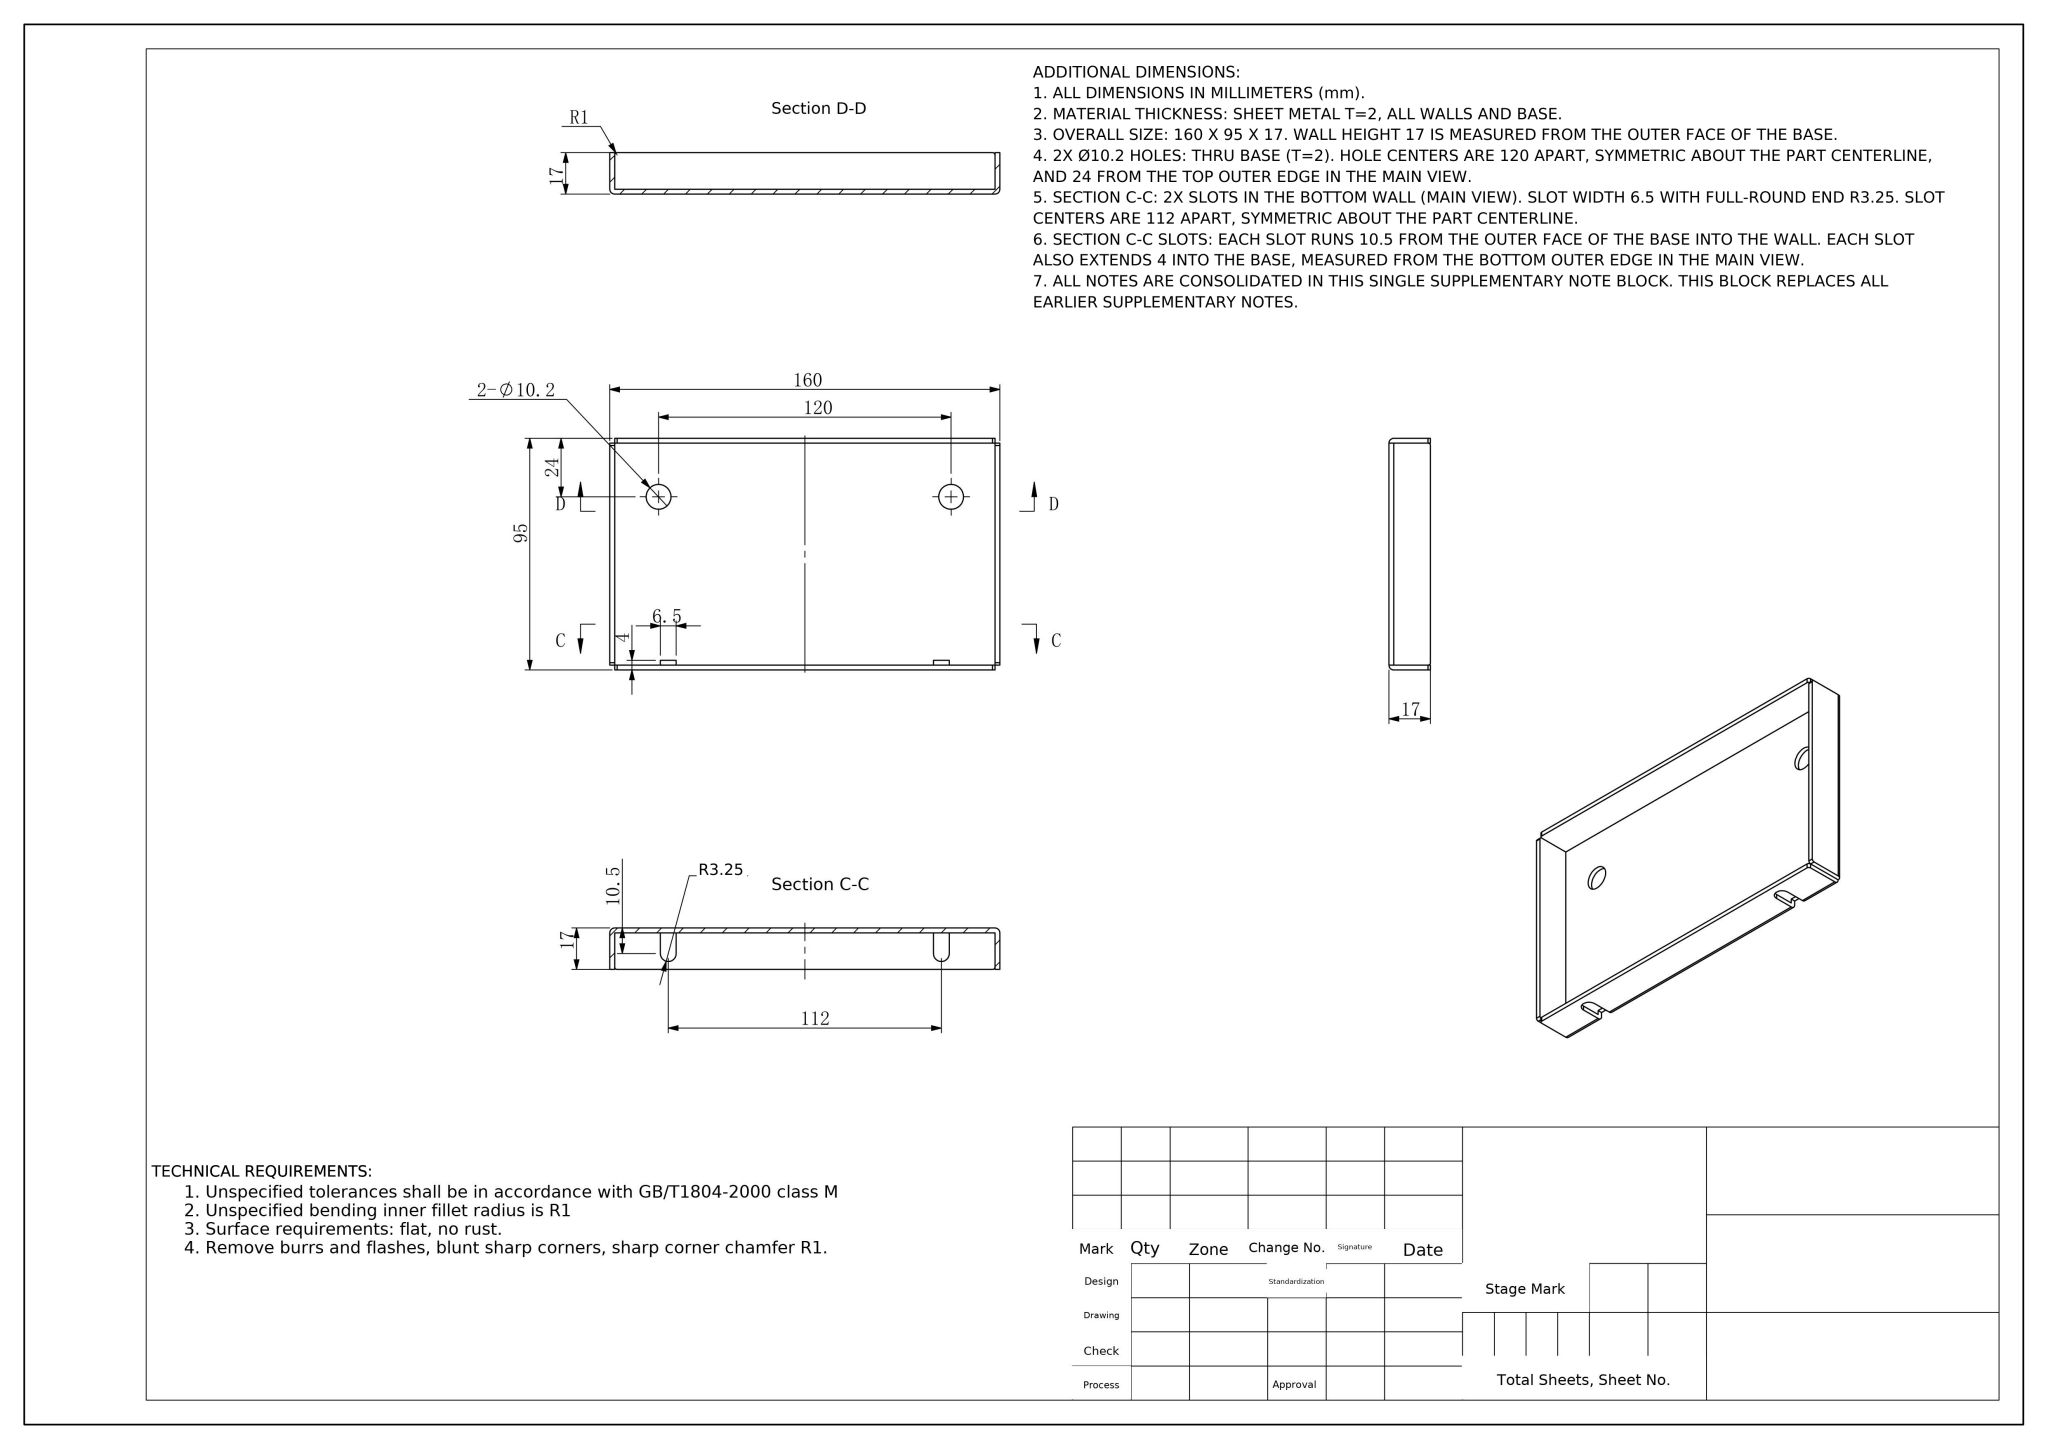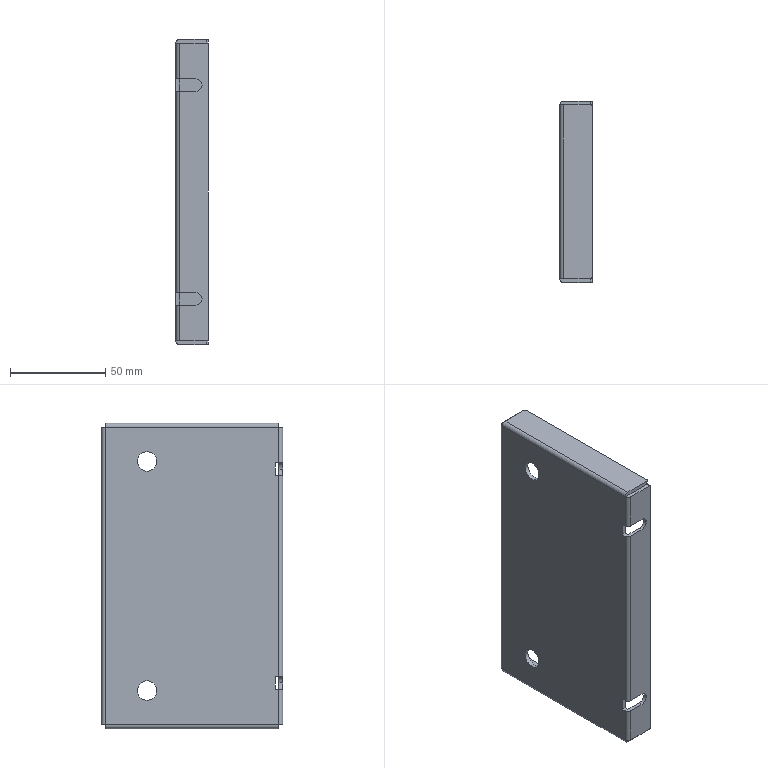Part | NX | mm | 1 solid | 64 faces | box 17 x 95 x 160 mm | volume 44052 mm3 | plane 36 | cylinder 28 | commonest cylinder face diameters 2 x8 4.004 x6 0.004 x6 10.2 x4 6.5 x4